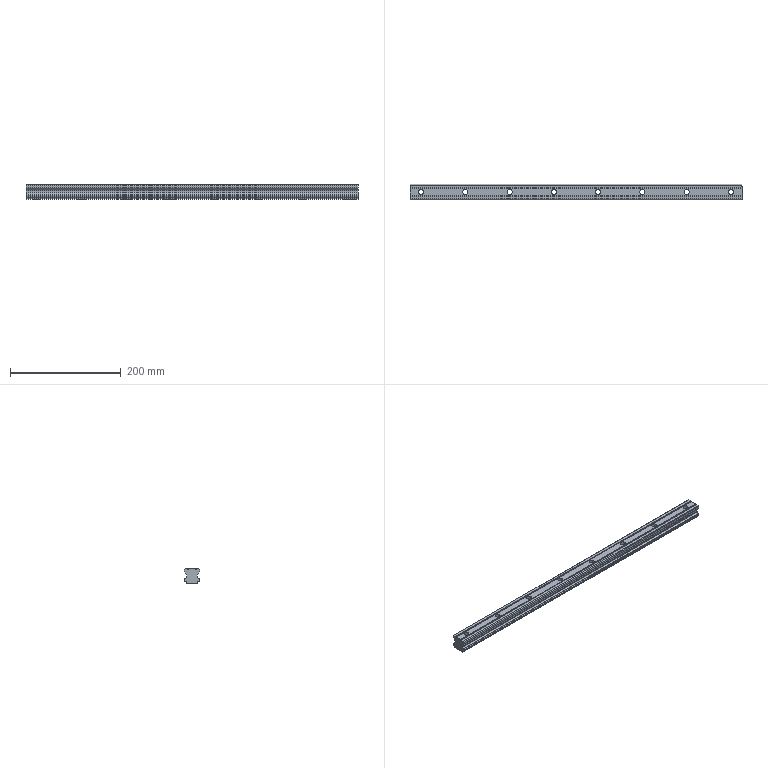Component | SolidWorks | GuideRailHGL30CA-600-3 | 1 solid | 92 faces | volume 346048 mm3 | cylinder 54 | plane 38 | commonest cylinder face diameters 14 x16 9 x16 1.2 x12 1.6 x6 5.66 x4